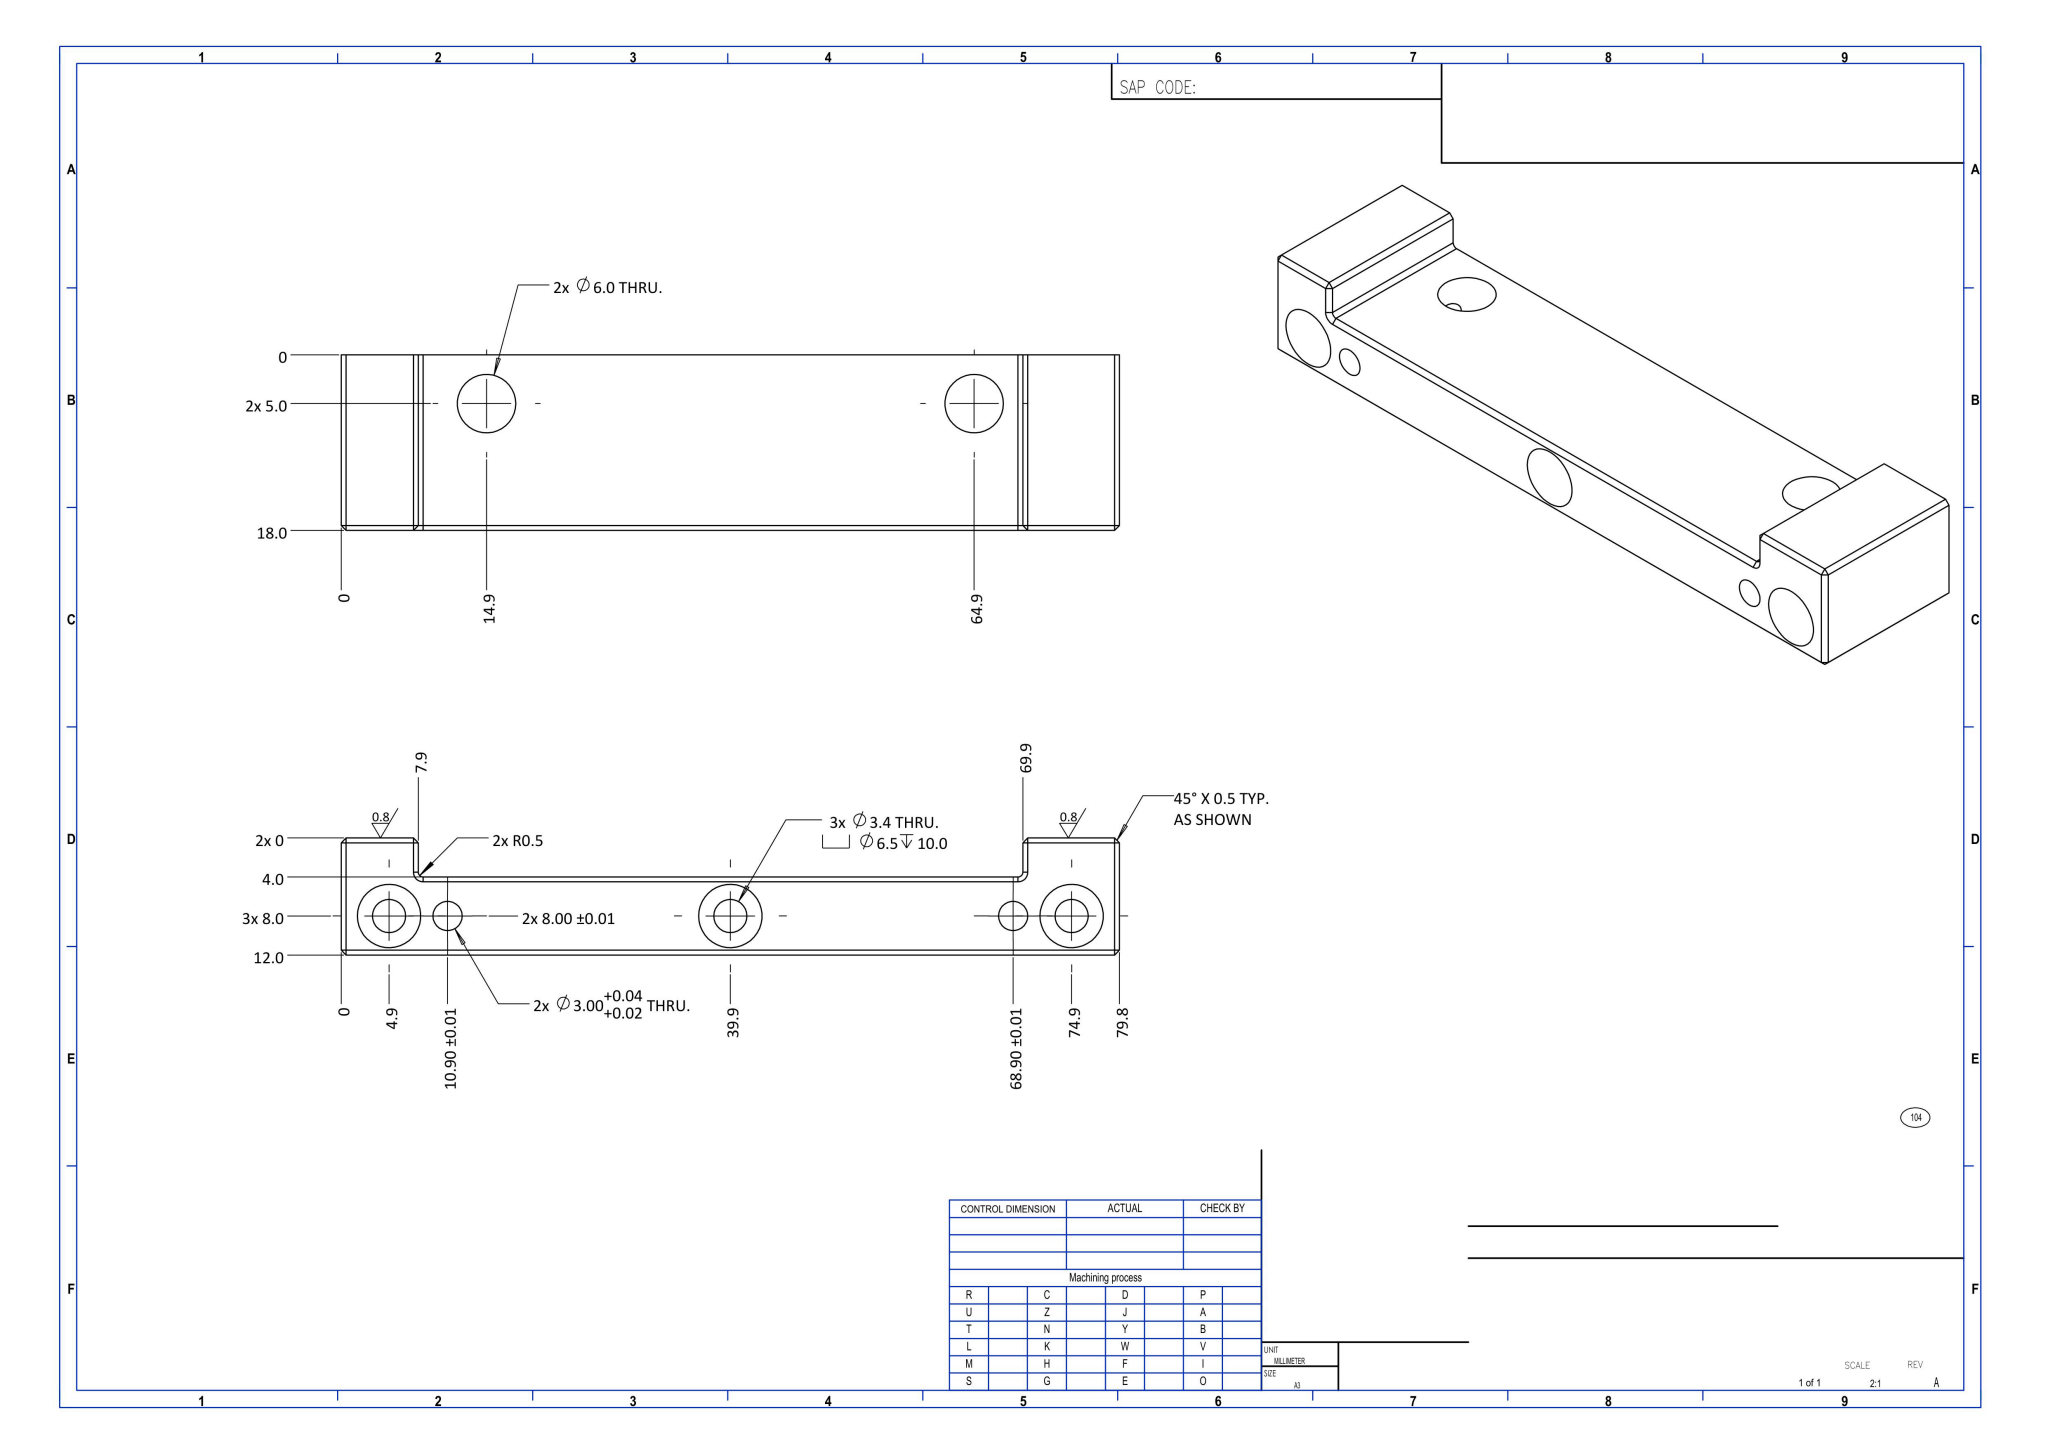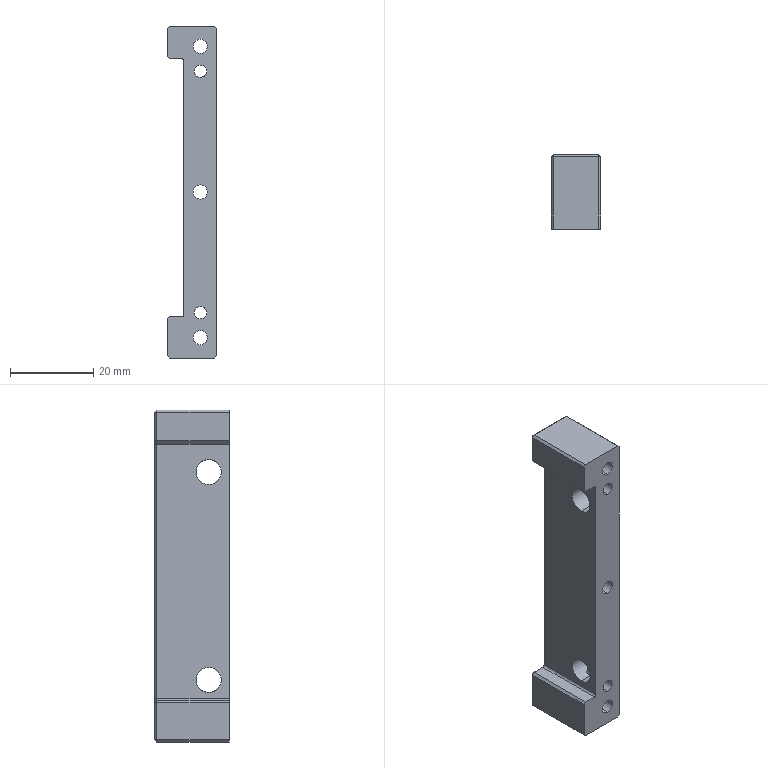Part | NX | mm | 1 solid | 57 faces | box 12 x 18 x 79.8 mm | volume 10821 mm3 | plane 33 | cylinder 22 | cone 2 | commonest cylinder face diameters 6.5 x6 3.4 x6 3 x4 6 x4 1 x2